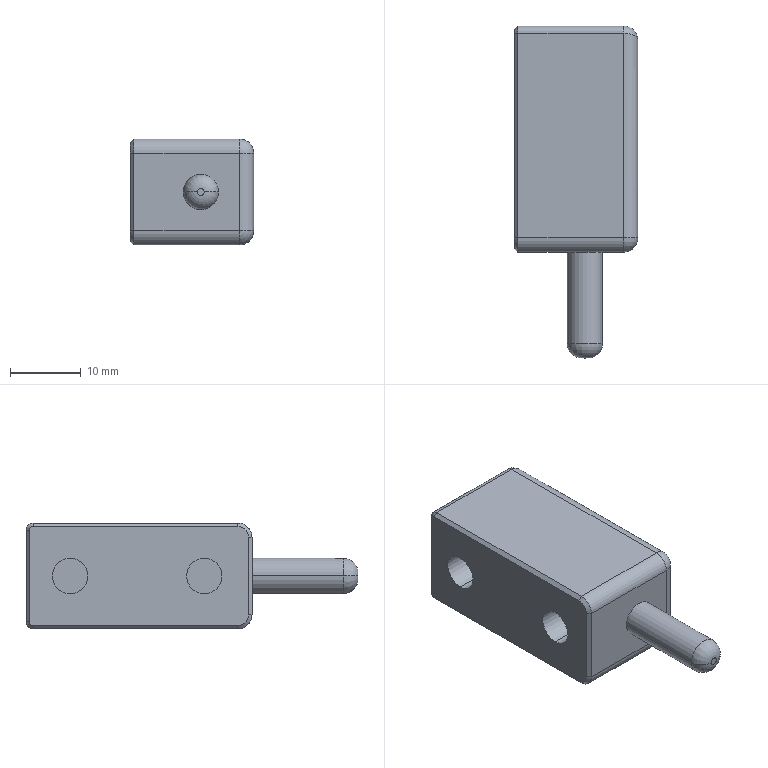Component | SolidWorks | LeftDoorPanelAssembly-1_CL203-2-A-1 | 1 solid | 37 faces | box 17.5 x 47 x 15 mm | volume 7950 mm3 | cylinder 14 | plane 13 | cone 4 | torus 2 | spline 2 | sphere 2 | commonest cylinder face diameters 5 x6 4 x6 2 x2
STEP:
#1=COLOUR_RGB('',0.7922,0.8196,0.9333);
#2=FILL_AREA_STYLE_COLOUR('',#1);
#3=FILL_AREA_STYLE('',(#2));
#4=SURFACE_STYLE_FILL_AREA(#3);
#5=SURFACE_SIDE_STYLE('',(#4));
#6=SURFACE_STYLE_USAGE(.BOTH.,#5);
#7=PRESENTATION_STYLE_ASSIGNMENT((#6));
#8=CARTESIAN_POINT('',(20.575,-3.877,-2.386));
#9=VERTEX_POINT('',#8);
#10=CARTESIAN_POINT('',(20.378,-3.877,-2.386));
#11=VERTEX_POINT('',#10);
#12=CARTESIAN_POINT('',(20.477,-3.877,-2.386));
#13=DIRECTION('',(-0.,1.,0.));
#14=DIRECTION('',(-1.,-0.,-0.));
#15=AXIS2_PLACEMENT_3D('',#12,#13,#14);
#16=CIRCLE('',#15,0.09843);
#17=EDGE_CURVE('',#9,#11,#16,.T.);
#18=ORIENTED_EDGE('',*,*,#17,.F.);
#19=CARTESIAN_POINT('',(20.496,-3.956,-2.386));
#20=VERTEX_POINT('',#19);
#21=CARTESIAN_POINT('',(20.496,-3.877,-2.386));
#22=DIRECTION('',(0.,0.,-1.));
#23=DIRECTION('',(-1.,0.,-0.));
#24=AXIS2_PLACEMENT_3D('',#21,#22,#23);
#25=CIRCLE('',#24,0.07874);
#26=EDGE_CURVE('',#9,#20,#25,.T.);
#27=ORIENTED_EDGE('',*,*,#26,.T.);
#28=CARTESIAN_POINT('',(20.457,-3.956,-2.386));
#29=VERTEX_POINT('',#28);
#30=CARTESIAN_POINT('',(20.477,-3.956,-2.386));
#31=DIRECTION('',(0.,-1.,-0.));
#32=DIRECTION('',(-1.,0.,-0.));
#33=AXIS2_PLACEMENT_3D('',#30,#31,#32);
#34=CIRCLE('',#33,0.01969);
#35=EDGE_CURVE('',#29,#20,#34,.T.);
#36=ORIENTED_EDGE('',*,*,#35,.F.);
#37=CARTESIAN_POINT('',(20.457,-3.877,-2.386));
#38=DIRECTION('',(-0.,-0.,1.));
#39=DIRECTION('',(1.,0.,0.));
#40=AXIS2_PLACEMENT_3D('',#37,#38,#39);
#41=CIRCLE('',#40,0.07874);
#42=EDGE_CURVE('',#11,#29,#41,.T.);
#43=ORIENTED_EDGE('',*,*,#42,.F.);
#44=EDGE_LOOP('',(#18,#27,#36,#43));
#45=FACE_OUTER_BOUND('',#44,.T.);
#46=CARTESIAN_POINT('',(20.477,-3.877,-2.386));
#47=DIRECTION('',(0.,-1.,-0.));
#48=DIRECTION('',(-1.,-0.,-0.));
#49=AXIS2_PLACEMENT_3D('',#46,#47,#48);
#50=TOROIDAL_SURFACE('',#49,0.01969,0.07874);
#51=ADVANCED_FACE('',(#45),#50,.T.);
#52=ORIENTED_EDGE('',*,*,#17,.T.);
#53=CARTESIAN_POINT('',(20.378,-3.365,-2.386));
#54=VERTEX_POINT('',#53);
#55=CARTESIAN_POINT('',(20.378,-3.956,-2.386));
#56=DIRECTION('',(-0.,1.,0.));
#57=VECTOR('',#56,39.37);
#58=LINE('',#55,#57);
#59=EDGE_CURVE('',#11,#54,#58,.T.);
#60=ORIENTED_EDGE('',*,*,#59,.T.);
#61=CARTESIAN_POINT('',(20.575,-3.365,-2.386));
#62=VERTEX_POINT('',#61);
#63=CARTESIAN_POINT('',(20.477,-3.365,-2.386));
#64=DIRECTION('',(0.,-1.,-0.));
#65=DIRECTION('',(1.,0.,0.));
#66=AXIS2_PLACEMENT_3D('',#63,#64,#65);
#67=CIRCLE('',#66,0.09843);
#68=EDGE_CURVE('',#54,#62,#67,.T.);
#69=ORIENTED_EDGE('',*,*,#68,.T.);
#70=CARTESIAN_POINT('',(20.575,-3.956,-2.386));
#71=DIRECTION('',(-0.,1.,0.));
#72=VECTOR('',#71,39.37);
#73=LINE('',#70,#72);
#74=EDGE_CURVE('',#9,#62,#73,.T.);
#75=ORIENTED_EDGE('',*,*,#74,.F.);
#76=EDGE_LOOP('',(#52,#60,#69,#75));
#77=FACE_OUTER_BOUND('',#76,.T.);
#78=CARTESIAN_POINT('',(20.477,-3.956,-2.386));
#79=DIRECTION('',(-0.,1.,0.));
#80=DIRECTION('',(1.,0.,0.));
#81=AXIS2_PLACEMENT_3D('',#78,#79,#80);
#82=CYLINDRICAL_SURFACE('',#81,0.09843);
#83=ADVANCED_FACE('',(#77),#82,.T.);
#84=CARTESIAN_POINT('',(20.083,-3.1,-2.287));
#85=VERTEX_POINT('',#84);
#86=CARTESIAN_POINT('',(20.083,-3.1,-2.484));
#87=VERTEX_POINT('',#86);
#88=CARTESIAN_POINT('',(20.083,-3.1,-2.386));
#89=DIRECTION('',(-1.,-0.,-0.));
#90=DIRECTION('',(0.,0.,-1.));
#91=AXIS2_PLACEMENT_3D('',#88,#89,#90);
#92=CIRCLE('',#91,0.09843);
#93=EDGE_CURVE('',#85,#87,#92,.T.);
#94=ORIENTED_EDGE('',*,*,#93,.T.);
#95=CARTESIAN_POINT('',(20.693,-3.1,-2.484));
#96=VERTEX_POINT('',#95);
#97=CARTESIAN_POINT('',(20.083,-3.1,-2.484));
#98=DIRECTION('',(1.,0.,0.));
#99=VECTOR('',#98,39.37);
#100=LINE('',#97,#99);
#101=EDGE_CURVE('',#87,#96,#100,.T.);
#102=ORIENTED_EDGE('',*,*,#101,.T.);
#103=CARTESIAN_POINT('',(20.693,-3.1,-2.287));
#104=VERTEX_POINT('',#103);
#105=CARTESIAN_POINT('',(20.693,-3.1,-2.386));
#106=DIRECTION('',(1.,0.,0.));
#107=DIRECTION('',(0.,-0.,1.));
#108=AXIS2_PLACEMENT_3D('',#105,#106,#107);
#109=CIRCLE('',#108,0.09843);
#110=EDGE_CURVE('',#96,#104,#109,.T.);
#111=ORIENTED_EDGE('',*,*,#110,.T.);
#112=CARTESIAN_POINT('',(20.083,-3.1,-2.287));
#113=DIRECTION('',(1.,0.,0.));
#114=VECTOR('',#113,39.37);
#115=LINE('',#112,#114);
#116=EDGE_CURVE('',#85,#104,#115,.T.);
#117=ORIENTED_EDGE('',*,*,#116,.F.);
#118=EDGE_LOOP('',(#94,#102,#111,#117));
#119=FACE_OUTER_BOUND('',#118,.T.);
#120=CARTESIAN_POINT('',(20.083,-3.1,-2.386));
#121=DIRECTION('',(1.,0.,0.));
#122=DIRECTION('',(0.,-0.,1.));
#123=AXIS2_PLACEMENT_3D('',#120,#121,#122);
#124=CYLINDRICAL_SURFACE('',#123,0.09843);
#125=ADVANCED_FACE('',(#119),#124,.F.);
#126=CARTESIAN_POINT('',(20.083,-2.352,-2.287));
#127=VERTEX_POINT('',#126);
#128=CARTESIAN_POINT('',(20.083,-2.352,-2.484));
#129=VERTEX_POINT('',#128);
#130=CARTESIAN_POINT('',(20.083,-2.352,-2.386));
#131=DIRECTION('',(-1.,-0.,-0.));
#132=DIRECTION('',(0.,0.,-1.));
#133=AXIS2_PLACEMENT_3D('',#130,#131,#132);
#134=CIRCLE('',#133,0.09843);
#135=EDGE_CURVE('',#127,#129,#134,.T.);
#136=ORIENTED_EDGE('',*,*,#135,.T.);
#137=CARTESIAN_POINT('',(20.693,-2.352,-2.484));
#138=VERTEX_POINT('',#137);
#139=CARTESIAN_POINT('',(20.083,-2.352,-2.484));
#140=DIRECTION('',(1.,0.,0.));
#141=VECTOR('',#140,39.37);
#142=LINE('',#139,#141);
#143=EDGE_CURVE('',#129,#138,#142,.T.);
#144=ORIENTED_EDGE('',*,*,#143,.T.);
#145=CARTESIAN_POINT('',(20.693,-2.352,-2.287));
#146=VERTEX_POINT('',#145);
#147=CARTESIAN_POINT('',(20.693,-2.352,-2.386));
#148=DIRECTION('',(1.,0.,0.));
#149=DIRECTION('',(0.,-0.,1.));
#150=AXIS2_PLACEMENT_3D('',#147,#148,#149);
#151=CIRCLE('',#150,0.09843);
#152=EDGE_CURVE('',#138,#146,#151,.T.);
#153=ORIENTED_EDGE('',*,*,#152,.T.);
#154=CARTESIAN_POINT('',(20.083,-2.352,-2.287));
#155=DIRECTION('',(1.,0.,0.));
#156=VECTOR('',#155,39.37);
#157=LINE('',#154,#156);
#158=EDGE_CURVE('',#127,#146,#157,.T.);
#159=ORIENTED_EDGE('',*,*,#158,.F.);
#160=EDGE_LOOP('',(#136,#144,#153,#159));
#161=FACE_OUTER_BOUND('',#160,.T.);
#162=CARTESIAN_POINT('',(20.083,-2.352,-2.386));
#163=DIRECTION('',(1.,0.,0.));
#164=DIRECTION('',(0.,-0.,1.));
#165=AXIS2_PLACEMENT_3D('',#162,#163,#164);
#166=CYLINDRICAL_SURFACE('',#165,0.09843);
#167=ADVANCED_FACE('',(#161),#166,.F.);
#168=ORIENTED_EDGE('',*,*,#143,.F.);
#169=CARTESIAN_POINT('',(20.083,-2.352,-2.386));
#170=DIRECTION('',(-1.,-0.,-0.));
#171=DIRECTION('',(0.,0.,-1.));
#172=AXIS2_PLACEMENT_3D('',#169,#170,#171);
#173=CIRCLE('',#172,0.09843);
#174=EDGE_CURVE('',#129,#127,#173,.T.);
#175=ORIENTED_EDGE('',*,*,#174,.T.);
#176=ORIENTED_EDGE('',*,*,#158,.T.);
#177=CARTESIAN_POINT('',(20.693,-2.352,-2.386));
#178=DIRECTION('',(1.,0.,0.));
#179=DIRECTION('',(0.,-0.,1.));
#180=AXIS2_PLACEMENT_3D('',#177,#178,#179);
#181=CIRCLE('',#180,0.09843);
#182=EDGE_CURVE('',#146,#138,#181,.T.);
#183=ORIENTED_EDGE('',*,*,#182,.T.);
#184=EDGE_LOOP('',(#168,#175,#176,#183));
#185=FACE_OUTER_BOUND('',#184,.T.);
#186=CARTESIAN_POINT('',(20.083,-2.352,-2.386));
#187=DIRECTION('',(1.,0.,0.));
#188=DIRECTION('',(0.,-0.,1.));
#189=AXIS2_PLACEMENT_3D('',#186,#187,#188);
#190=CYLINDRICAL_SURFACE('',#189,0.09843);
#191=ADVANCED_FACE('',(#185),#190,.F.);
#192=ORIENTED_EDGE('',*,*,#101,.F.);
#193=CARTESIAN_POINT('',(20.083,-3.1,-2.386));
#194=DIRECTION('',(-1.,-0.,-0.));
#195=DIRECTION('',(0.,0.,-1.));
#196=AXIS2_PLACEMENT_3D('',#193,#194,#195);
#197=CIRCLE('',#196,0.09843);
#198=EDGE_CURVE('',#87,#85,#197,.T.);
#199=ORIENTED_EDGE('',*,*,#198,.T.);
#200=ORIENTED_EDGE('',*,*,#116,.T.);
#201=CARTESIAN_POINT('',(20.693,-3.1,-2.386));
#202=DIRECTION('',(1.,0.,0.));
#203=DIRECTION('',(0.,-0.,1.));
#204=AXIS2_PLACEMENT_3D('',#201,#202,#203);
#205=CIRCLE('',#204,0.09843);
#206=EDGE_CURVE('',#104,#96,#205,.T.);
#207=ORIENTED_EDGE('',*,*,#206,.T.);
#208=EDGE_LOOP('',(#192,#199,#200,#207));
#209=FACE_OUTER_BOUND('',#208,.T.);
#210=CARTESIAN_POINT('',(20.083,-3.1,-2.386));
#211=DIRECTION('',(1.,0.,0.));
#212=DIRECTION('',(0.,-0.,1.));
#213=AXIS2_PLACEMENT_3D('',#210,#211,#212);
#214=CYLINDRICAL_SURFACE('',#213,0.09843);
#215=ADVANCED_FACE('',(#209),#214,.F.);
#216=CARTESIAN_POINT('',(20.693,-3.365,-2.169));
#217=VERTEX_POINT('',#216);
#218=CARTESIAN_POINT('',(20.103,-3.365,-2.169));
#219=VERTEX_POINT('',#218);
#220=CARTESIAN_POINT('',(20.083,-3.365,-2.169));
#221=DIRECTION('',(-1.,-0.,-0.));
#222=VECTOR('',#221,39.37);
#223=LINE('',#220,#222);
#224=EDGE_CURVE('',#217,#219,#223,.T.);
#225=ORIENTED_EDGE('',*,*,#224,.T.);
#226=CARTESIAN_POINT('',(20.103,-3.365,-2.602));
#227=VERTEX_POINT('',#226);
#228=CARTESIAN_POINT('',(20.103,-3.365,-2.602));
#229=DIRECTION('',(0.,0.,-1.));
#230=VECTOR('',#229,39.37);
#231=LINE('',#228,#230);
#232=EDGE_CURVE('',#219,#227,#231,.T.);
#233=ORIENTED_EDGE('',*,*,#232,.T.);
#234=CARTESIAN_POINT('',(20.693,-3.365,-2.602));
#235=VERTEX_POINT('',#234);
#236=CARTESIAN_POINT('',(20.083,-3.365,-2.602));
#237=DIRECTION('',(1.,0.,0.));
#238=VECTOR('',#237,39.37);
#239=LINE('',#236,#238);
#240=EDGE_CURVE('',#227,#235,#239,.T.);
#241=ORIENTED_EDGE('',*,*,#240,.T.);
#242=CARTESIAN_POINT('',(20.693,-3.365,-2.091));
#243=DIRECTION('',(-0.,-0.,1.));
#244=VECTOR('',#243,39.37);
#245=LINE('',#242,#244);
#246=EDGE_CURVE('',#235,#217,#245,.T.);
#247=ORIENTED_EDGE('',*,*,#246,.T.);
#248=EDGE_LOOP('',(#225,#233,#241,#247));
#249=FACE_OUTER_BOUND('',#248,.T.);
#250=CARTESIAN_POINT('',(20.477,-3.365,-2.386));
#251=DIRECTION('',(0.,-1.,-0.));
#252=DIRECTION('',(1.,0.,0.));
#253=AXIS2_PLACEMENT_3D('',#250,#251,#252);
#254=CIRCLE('',#253,0.09843);
#255=EDGE_CURVE('',#62,#54,#254,.T.);
#256=ORIENTED_EDGE('',*,*,#255,.F.);
#257=ORIENTED_EDGE('',*,*,#68,.F.);
#258=EDGE_LOOP('',(#256,#257));
#259=FACE_BOUND('',#258,.T.);
#260=CARTESIAN_POINT('',(20.083,-3.365,-2.091));
#261=DIRECTION('',(-0.,1.,0.));
#262=DIRECTION('',(1.,0.,0.));
#263=AXIS2_PLACEMENT_3D('',#260,#261,#262);
#264=PLANE('',#263);
#265=ADVANCED_FACE('',(#249,#259),#264,.F.);
#266=CARTESIAN_POINT('',(20.083,-3.346,-2.169));
#267=VERTEX_POINT('',#266);
#268=CARTESIAN_POINT('',(20.083,-3.287,-2.11));
#269=VERTEX_POINT('',#268);
#270=CARTESIAN_POINT('',(20.083,-3.287,-2.169));
#271=DIRECTION('',(-1.,-0.,-0.));
#272=DIRECTION('',(0.,0.,-1.));
#273=AXIS2_PLACEMENT_3D('',#270,#271,#272);
#274=CIRCLE('',#273,0.05906);
#275=EDGE_CURVE('',#267,#269,#274,.T.);
#276=ORIENTED_EDGE('',*,*,#275,.T.);
#277=CARTESIAN_POINT('',(20.083,-2.145,-2.11));
#278=VERTEX_POINT('',#277);
#279=CARTESIAN_POINT('',(20.083,-2.145,-2.11));
#280=DIRECTION('',(-0.,1.,0.));
#281=VECTOR('',#280,39.37);
#282=LINE('',#279,#281);
#283=EDGE_CURVE('',#269,#278,#282,.T.);
#284=ORIENTED_EDGE('',*,*,#283,.T.);
#285=CARTESIAN_POINT('',(20.083,-2.125,-2.13));
#286=VERTEX_POINT('',#285);
#287=CARTESIAN_POINT('',(20.083,-2.145,-2.13));
#288=DIRECTION('',(-1.,-0.,-0.));
#289=DIRECTION('',(0.,0.,-1.));
#290=AXIS2_PLACEMENT_3D('',#287,#288,#289);
#291=CIRCLE('',#290,0.01969);
#292=EDGE_CURVE('',#278,#286,#291,.T.);
#293=ORIENTED_EDGE('',*,*,#292,.T.);
#294=CARTESIAN_POINT('',(20.083,-2.125,-2.642));
#295=VERTEX_POINT('',#294);
#296=CARTESIAN_POINT('',(20.083,-2.125,-2.642));
#297=DIRECTION('',(0.,0.,-1.));
#298=VECTOR('',#297,39.37);
#299=LINE('',#296,#298);
#300=EDGE_CURVE('',#286,#295,#299,.T.);
#301=ORIENTED_EDGE('',*,*,#300,.T.);
#302=CARTESIAN_POINT('',(20.083,-2.145,-2.661));
#303=VERTEX_POINT('',#302);
#304=CARTESIAN_POINT('',(20.083,-2.145,-2.642));
#305=DIRECTION('',(-1.,-0.,-0.));
#306=DIRECTION('',(0.,0.,-1.));
#307=AXIS2_PLACEMENT_3D('',#304,#305,#306);
#308=CIRCLE('',#307,0.01969);
#309=EDGE_CURVE('',#295,#303,#308,.T.);
#310=ORIENTED_EDGE('',*,*,#309,.T.);
#311=CARTESIAN_POINT('',(20.083,-3.287,-2.661));
#312=VERTEX_POINT('',#311);
#313=CARTESIAN_POINT('',(20.083,-3.287,-2.661));
#314=DIRECTION('',(0.,-1.,-0.));
#315=VECTOR('',#314,39.37);
#316=LINE('',#313,#315);
#317=EDGE_CURVE('',#303,#312,#316,.T.);
#318=ORIENTED_EDGE('',*,*,#317,.T.);
#319=CARTESIAN_POINT('',(20.083,-3.346,-2.602));
#320=VERTEX_POINT('',#319);
#321=CARTESIAN_POINT('',(20.083,-3.287,-2.602));
#322=DIRECTION('',(-1.,-0.,-0.));
#323=DIRECTION('',(0.,0.,-1.));
#324=AXIS2_PLACEMENT_3D('',#321,#322,#323);
#325=CIRCLE('',#324,0.05906);
#326=EDGE_CURVE('',#312,#320,#325,.T.);
#327=ORIENTED_EDGE('',*,*,#326,.T.);
#328=CARTESIAN_POINT('',(20.083,-3.346,-2.169));
#329=DIRECTION('',(-0.,-0.,1.));
#330=VECTOR('',#329,39.37);
#331=LINE('',#328,#330);
#332=EDGE_CURVE('',#320,#267,#331,.T.);
#333=ORIENTED_EDGE('',*,*,#332,.T.);
#334=EDGE_LOOP('',(#276,#284,#293,#301,#310,#318,#327,#333));
#335=FACE_OUTER_BOUND('',#334,.T.);
#336=ORIENTED_EDGE('',*,*,#93,.F.);
#337=ORIENTED_EDGE('',*,*,#198,.F.);
#338=EDGE_LOOP('',(#336,#337));
#339=FACE_BOUND('',#338,.T.);
#340=ORIENTED_EDGE('',*,*,#135,.F.);
#341=ORIENTED_EDGE('',*,*,#174,.F.);
#342=EDGE_LOOP('',(#340,#341));
#343=FACE_BOUND('',#342,.T.);
#344=CARTESIAN_POINT('',(20.083,-2.145,-2.642));
#345=DIRECTION('',(-1.,-0.,-0.));
#346=DIRECTION('',(0.,0.,-1.));
#347=AXIS2_PLACEMENT_3D('',#344,#345,#346);
#348=PLANE('',#347);
#349=ADVANCED_FACE('',(#335,#339,#343),#348,.T.);
#350=CARTESIAN_POINT('',(20.772,-2.184,-2.169));
#351=VERTEX_POINT('',#350);
#352=CARTESIAN_POINT('',(20.772,-3.287,-2.169));
#353=VERTEX_POINT('',#352);
#354=CARTESIAN_POINT('',(20.772,-2.145,-2.169));
#355=DIRECTION('',(0.,-1.,-0.));
#356=VECTOR('',#355,39.37);
#357=LINE('',#354,#356);
#358=EDGE_CURVE('',#351,#353,#357,.T.);
#359=ORIENTED_EDGE('',*,*,#358,.T.);
#360=CARTESIAN_POINT('',(20.772,-3.287,-2.602));
#361=VERTEX_POINT('',#360);
#362=CARTESIAN_POINT('',(20.772,-3.287,-2.642));
#363=DIRECTION('',(0.,0.,-1.));
#364=VECTOR('',#363,39.37);
#365=LINE('',#362,#364);
#366=EDGE_CURVE('',#353,#361,#365,.T.);
#367=ORIENTED_EDGE('',*,*,#366,.T.);
#368=CARTESIAN_POINT('',(20.772,-2.184,-2.602));
#369=VERTEX_POINT('',#368);
#370=CARTESIAN_POINT('',(20.772,-2.145,-2.602));
#371=DIRECTION('',(-0.,1.,0.));
#372=VECTOR('',#371,39.37);
#373=LINE('',#370,#372);
#374=EDGE_CURVE('',#361,#369,#373,.T.);
#375=ORIENTED_EDGE('',*,*,#374,.T.);
#376=CARTESIAN_POINT('',(20.772,-2.184,-2.642));
#377=DIRECTION('',(-0.,-0.,1.));
#378=VECTOR('',#377,39.37);
#379=LINE('',#376,#378);
#380=EDGE_CURVE('',#369,#351,#379,.T.);
#381=ORIENTED_EDGE('',*,*,#380,.T.);
#382=EDGE_LOOP('',(#359,#367,#375,#381));
#383=FACE_OUTER_BOUND('',#382,.T.);
#384=CARTESIAN_POINT('',(20.772,-2.145,-2.642));
#385=DIRECTION('',(-1.,-0.,-0.));
#386=DIRECTION('',(0.,0.,-1.));
#387=AXIS2_PLACEMENT_3D('',#384,#385,#386);
#388=PLANE('',#387);
#389=ADVANCED_FACE('',(#383),#388,.F.);
#390=CARTESIAN_POINT('',(20.103,-2.145,-2.091));
#391=VERTEX_POINT('',#390);
#392=CARTESIAN_POINT('',(20.693,-2.145,-2.091));
#393=VERTEX_POINT('',#392);
#394=CARTESIAN_POINT('',(20.083,-2.145,-2.091));
#395=DIRECTION('',(1.,0.,0.));
#396=VECTOR('',#395,39.37);
#397=LINE('',#394,#396);
#398=EDGE_CURVE('',#391,#393,#397,.T.);
#399=ORIENTED_EDGE('',*,*,#398,.F.);
#400=CARTESIAN_POINT('',(20.103,-3.287,-2.091));
#401=VERTEX_POINT('',#400);
#402=CARTESIAN_POINT('',(20.103,-3.287,-2.091));
#403=DIRECTION('',(0.,-1.,-0.));
#404=VECTOR('',#403,39.37);
#405=LINE('',#402,#404);
#406=EDGE_CURVE('',#391,#401,#405,.T.);
#407=ORIENTED_EDGE('',*,*,#406,.T.);
#408=CARTESIAN_POINT('',(20.693,-3.287,-2.091));
#409=VERTEX_POINT('',#408);
#410=CARTESIAN_POINT('',(20.083,-3.287,-2.091));
#411=DIRECTION('',(1.,0.,0.));
#412=VECTOR('',#411,39.37);
#413=LINE('',#410,#412);
#414=EDGE_CURVE('',#401,#409,#413,.T.);
#415=ORIENTED_EDGE('',*,*,#414,.T.);
#416=CARTESIAN_POINT('',(20.693,-3.365,-2.091));
#417=DIRECTION('',(-0.,1.,0.));
#418=VECTOR('',#417,39.37);
#419=LINE('',#416,#418);
#420=EDGE_CURVE('',#409,#393,#419,.T.);
#421=ORIENTED_EDGE('',*,*,#420,.T.);
#422=EDGE_LOOP('',(#399,#407,#415,#421));
#423=FACE_OUTER_BOUND('',#422,.T.);
#424=CARTESIAN_POINT('',(20.083,-3.365,-2.091));
#425=DIRECTION('',(0.,0.,-1.));
#426=DIRECTION('',(1.,0.,0.));
#427=AXIS2_PLACEMENT_3D('',#424,#425,#426);
#428=PLANE('',#427);
#429=ADVANCED_FACE('',(#423),#428,.F.);
#430=CARTESIAN_POINT('',(20.103,-2.105,-2.13));
#431=VERTEX_POINT('',#430);
#432=CARTESIAN_POINT('',(20.693,-2.105,-2.13));
#433=VERTEX_POINT('',#432);
#434=CARTESIAN_POINT('',(20.083,-2.105,-2.13));
#435=DIRECTION('',(1.,0.,0.));
#436=VECTOR('',#435,39.37);
#437=LINE('',#434,#436);
#438=EDGE_CURVE('',#431,#433,#437,.T.);
#439=ORIENTED_EDGE('',*,*,#438,.F.);
#440=CARTESIAN_POINT('',(20.103,-2.145,-2.13));
#441=DIRECTION('',(1.,0.,0.));
#442=DIRECTION('',(0.,0.,-1.));
#443=AXIS2_PLACEMENT_3D('',#440,#441,#442);
#444=CIRCLE('',#443,0.03937);
#445=EDGE_CURVE('',#431,#391,#444,.T.);
#446=ORIENTED_EDGE('',*,*,#445,.T.);
#447=ORIENTED_EDGE('',*,*,#398,.T.);
#448=CARTESIAN_POINT('',(20.693,-2.145,-2.13));
#449=DIRECTION('',(-1.,-0.,-0.));
#450=DIRECTION('',(0.,0.,-1.));
#451=AXIS2_PLACEMENT_3D('',#448,#449,#450);
#452=CIRCLE('',#451,0.03937);
#453=EDGE_CURVE('',#393,#433,#452,.T.);
#454=ORIENTED_EDGE('',*,*,#453,.T.);
#455=EDGE_LOOP('',(#439,#446,#447,#454));
#456=FACE_OUTER_BOUND('',#455,.T.);
#457=CARTESIAN_POINT('',(20.083,-2.145,-2.13));
#458=DIRECTION('',(1.,0.,0.));
#459=DIRECTION('',(0.,-0.,1.));
#460=AXIS2_PLACEMENT_3D('',#457,#458,#459);
#461=CYLINDRICAL_SURFACE('',#460,0.03937);
#462=ADVANCED_FACE('',(#456),#461,.T.);
#463=CARTESIAN_POINT('',(20.103,-2.105,-2.642));
#464=VERTEX_POINT('',#463);
#465=CARTESIAN_POINT('',(20.693,-2.105,-2.642));
#466=VERTEX_POINT('',#465);
#467=CARTESIAN_POINT('',(20.083,-2.105,-2.642));
#468=DIRECTION('',(1.,0.,0.));
#469=VECTOR('',#468,39.37);
#470=LINE('',#467,#469);
#471=EDGE_CURVE('',#464,#466,#470,.T.);
#472=ORIENTED_EDGE('',*,*,#471,.F.);
#473=CARTESIAN_POINT('',(20.103,-2.105,-2.13));
#474=DIRECTION('',(-0.,-0.,1.));
#475=VECTOR('',#474,39.37);
#476=LINE('',#473,#475);
#477=EDGE_CURVE('',#464,#431,#476,.T.);
#478=ORIENTED_EDGE('',*,*,#477,.T.);
#479=ORIENTED_EDGE('',*,*,#438,.T.);
#480=CARTESIAN_POINT('',(20.693,-2.105,-2.13));
#481=DIRECTION('',(0.,0.,-1.));
#482=VECTOR('',#481,39.37);
#483=LINE('',#480,#482);
#484=EDGE_CURVE('',#433,#466,#483,.T.);
#485=ORIENTED_EDGE('',*,*,#484,.T.);
#486=EDGE_LOOP('',(#472,#478,#479,#485));
#487=FACE_OUTER_BOUND('',#486,.T.);
#488=CARTESIAN_POINT('',(20.083,-2.105,-2.13));
#489=DIRECTION('',(0.,-1.,-0.));
#490=DIRECTION('',(-1.,-0.,-0.));
#491=AXIS2_PLACEMENT_3D('',#488,#489,#490);
#492=PLANE('',#491);
#493=ADVANCED_FACE('',(#487),#492,.F.);
#494=CARTESIAN_POINT('',(20.103,-2.145,-2.681));
#495=VERTEX_POINT('',#494);
#496=CARTESIAN_POINT('',(20.693,-2.145,-2.681));
#497=VERTEX_POINT('',#496);
#498=CARTESIAN_POINT('',(20.083,-2.145,-2.681));
#499=DIRECTION('',(1.,0.,0.));
#500=VECTOR('',#499,39.37);
#501=LINE('',#498,#500);
#502=EDGE_CURVE('',#495,#497,#501,.T.);
#503=ORIENTED_EDGE('',*,*,#502,.F.);
#504=CARTESIAN_POINT('',(20.103,-2.145,-2.642));
#505=DIRECTION('',(1.,0.,0.));
#506=DIRECTION('',(0.,0.,-1.));
#507=AXIS2_PLACEMENT_3D('',#504,#505,#506);
#508=CIRCLE('',#507,0.03937);
#509=EDGE_CURVE('',#495,#464,#508,.T.);
#510=ORIENTED_EDGE('',*,*,#509,.T.);
#511=ORIENTED_EDGE('',*,*,#471,.T.);
#512=CARTESIAN_POINT('',(20.693,-2.145,-2.642));
#513=DIRECTION('',(-1.,-0.,-0.));
#514=DIRECTION('',(0.,0.,-1.));
#515=AXIS2_PLACEMENT_3D('',#512,#513,#514);
#516=CIRCLE('',#515,0.03937);
#517=EDGE_CURVE('',#466,#497,#516,.T.);
#518=ORIENTED_EDGE('',*,*,#517,.T.);
#519=EDGE_LOOP('',(#503,#510,#511,#518));
#520=FACE_OUTER_BOUND('',#519,.T.);
#521=CARTESIAN_POINT('',(20.083,-2.145,-2.642));
#522=DIRECTION('',(1.,0.,0.));
#523=DIRECTION('',(0.,-0.,1.));
#524=AXIS2_PLACEMENT_3D('',#521,#522,#523);
#525=CYLINDRICAL_SURFACE('',#524,0.03937);
#526=ADVANCED_FACE('',(#520),#525,.T.);
#527=CARTESIAN_POINT('',(20.693,-3.287,-2.681));
#528=VERTEX_POINT('',#527);
#529=CARTESIAN_POINT('',(20.103,-3.287,-2.681));
#530=VERTEX_POINT('',#529);
#531=CARTESIAN_POINT('',(20.083,-3.287,-2.681));
#532=DIRECTION('',(-1.,-0.,-0.));
#533=VECTOR('',#532,39.37);
#534=LINE('',#531,#533);
#535=EDGE_CURVE('',#528,#530,#534,.T.);
#536=ORIENTED_EDGE('',*,*,#535,.T.);
#537=CARTESIAN_POINT('',(20.103,-2.145,-2.681));
#538=DIRECTION('',(-0.,1.,0.));
#539=VECTOR('',#538,39.37);
#540=LINE('',#537,#539);
#541=EDGE_CURVE('',#530,#495,#540,.T.);
#542=ORIENTED_EDGE('',*,*,#541,.T.);
#543=ORIENTED_EDGE('',*,*,#502,.T.);
#544=CARTESIAN_POINT('',(20.693,-2.145,-2.681));
#545=DIRECTION('',(0.,-1.,-0.));
#546=VECTOR('',#545,39.37);
#547=LINE('',#544,#546);
#548=EDGE_CURVE('',#497,#528,#547,.T.);
#549=ORIENTED_EDGE('',*,*,#548,.T.);
#550=EDGE_LOOP('',(#536,#542,#543,#549));
#551=FACE_OUTER_BOUND('',#550,.T.);
#552=CARTESIAN_POINT('',(20.083,-2.145,-2.681));
#553=DIRECTION('',(-0.,-0.,1.));
#554=DIRECTION('',(-1.,-0.,-0.));
#555=AXIS2_PLACEMENT_3D('',#552,#553,#554);
#556=PLANE('',#555);
#557=ADVANCED_FACE('',(#551),#556,.F.);
#558=ORIENTED_EDGE('',*,*,#420,.F.);
#559=CARTESIAN_POINT('',(20.693,-3.287,-2.169));
#560=DIRECTION('',(-0.,1.,0.));
#561=DIRECTION('',(1.,0.,0.));
#562=AXIS2_PLACEMENT_3D('',#559,#560,#561);
#563=CIRCLE('',#562,0.07874);
#564=EDGE_CURVE('',#409,#353,#563,.T.);
#565=ORIENTED_EDGE('',*,*,#564,.T.);
#566=ORIENTED_EDGE('',*,*,#358,.F.);
#567=CARTESIAN_POINT('',(20.693,-2.145,-2.091));
#568=CARTESIAN_POINT('',(20.739,-2.145,-2.091));
#569=CARTESIAN_POINT('',(20.772,-2.161,-2.123));
#570=CARTESIAN_POINT('',(20.772,-2.184,-2.169));
#571=(BOUNDED_CURVE()B_SPLINE_CURVE(3,(#567,#568,#569,#570),.UNSPECIFIED.,.F.,.F.)B_SPLINE_CURVE_WITH_KNOTS((4,4),(0.,1.571),.UNSPECIFIED.)CURVE()GEOMETRIC_REPRESENTATION_ITEM()RATIONAL_B_SPLINE_CURVE((1.,0.8047,0.8047,1.))REPRESENTATION_ITEM(''));
#572=EDGE_CURVE('',#393,#351,#571,.T.);
#573=ORIENTED_EDGE('',*,*,#572,.F.);
#574=EDGE_LOOP('',(#558,#565,#566,#573));
#575=FACE_OUTER_BOUND('',#574,.T.);
#576=CARTESIAN_POINT('',(20.693,-3.365,-2.169));
#577=DIRECTION('',(-0.,1.,0.));
#578=DIRECTION('',(1.,0.,0.));
#579=AXIS2_PLACEMENT_3D('',#576,#577,#578);
#580=CYLINDRICAL_SURFACE('',#579,0.07874);
#581=ADVANCED_FACE('',(#575),#580,.T.);
#582=ORIENTED_EDGE('',*,*,#453,.F.);
#583=ORIENTED_EDGE('',*,*,#572,.T.);
#584=CARTESIAN_POINT('',(20.693,-2.105,-2.13));
#585=CARTESIAN_POINT('',(20.739,-2.105,-2.13));
#586=CARTESIAN_POINT('',(20.772,-2.138,-2.146));
#587=CARTESIAN_POINT('',(20.772,-2.184,-2.169));
#588=(BOUNDED_CURVE()B_SPLINE_CURVE(3,(#584,#585,#586,#587),.UNSPECIFIED.,.F.,.T.)B_SPLINE_CURVE_WITH_KNOTS((4,4),(0.,1.571),.UNSPECIFIED.)CURVE()GEOMETRIC_REPRESENTATION_ITEM()RATIONAL_B_SPLINE_CURVE((1.,0.8047,0.8047,1.))REPRESENTATION_ITEM(''));
#589=EDGE_CURVE('',#433,#351,#588,.T.);
#590=ORIENTED_EDGE('',*,*,#589,.F.);
#591=EDGE_LOOP('',(#582,#583,#590));
#592=FACE_OUTER_BOUND('',#591,.T.);
#593=CARTESIAN_POINT('',(20.693,-2.145,-2.091));
#594=CARTESIAN_POINT('',(20.693,-2.105,-2.091));
#595=CARTESIAN_POINT('',(20.693,-2.105,-2.13));
#596=CARTESIAN_POINT('',(20.698,-2.145,-2.091));
#597=CARTESIAN_POINT('',(20.701,-2.105,-2.091));
#598=CARTESIAN_POINT('',(20.698,-2.105,-2.13));
#599=CARTESIAN_POINT('',(20.704,-2.145,-2.091));
#600=CARTESIAN_POINT('',(20.709,-2.106,-2.092));
#601=CARTESIAN_POINT('',(20.704,-2.106,-2.13));
#602=CARTESIAN_POINT('',(20.714,-2.146,-2.093));
#603=CARTESIAN_POINT('',(20.723,-2.11,-2.095));
#604=CARTESIAN_POINT('',(20.714,-2.108,-2.131));
#605=CARTESIAN_POINT('',(20.719,-2.147,-2.095));
#606=CARTESIAN_POINT('',(20.729,-2.113,-2.098));
#607=CARTESIAN_POINT('',(20.719,-2.109,-2.132));
#608=CARTESIAN_POINT('',(20.728,-2.149,-2.099));
#609=CARTESIAN_POINT('',(20.74,-2.119,-2.104));
#610=CARTESIAN_POINT('',(20.728,-2.113,-2.134));
#611=CARTESIAN_POINT('',(20.733,-2.15,-2.101));
#612=CARTESIAN_POINT('',(20.745,-2.123,-2.108));
#613=CARTESIAN_POINT('',(20.733,-2.116,-2.135));
#614=CARTESIAN_POINT('',(20.741,-2.153,-2.107));
#615=CARTESIAN_POINT('',(20.752,-2.13,-2.115));
#616=CARTESIAN_POINT('',(20.741,-2.122,-2.138));
#617=CARTESIAN_POINT('',(20.745,-2.155,-2.11));
#618=CARTESIAN_POINT('',(20.756,-2.134,-2.119));
#619=CARTESIAN_POINT('',(20.745,-2.125,-2.14));
#620=CARTESIAN_POINT('',(20.756,-2.16,-2.121));
#621=CARTESIAN_POINT('',(20.763,-2.145,-2.13));
#622=CARTESIAN_POINT('',(20.756,-2.136,-2.145));
#623=CARTESIAN_POINT('',(20.762,-2.164,-2.13));
#624=CARTESIAN_POINT('',(20.767,-2.153,-2.138));
#625=CARTESIAN_POINT('',(20.762,-2.145,-2.149));
#626=CARTESIAN_POINT('',(20.77,-2.174,-2.149));
#627=CARTESIAN_POINT('',(20.771,-2.169,-2.154));
#628=CARTESIAN_POINT('',(20.77,-2.164,-2.159));
#629=CARTESIAN_POINT('',(20.772,-2.179,-2.159));
#630=CARTESIAN_POINT('',(20.772,-2.176,-2.162));
#631=CARTESIAN_POINT('',(20.772,-2.174,-2.164));
#632=CARTESIAN_POINT('',(20.772,-2.184,-2.169));
#633=CARTESIAN_POINT('',(20.772,-2.184,-2.169));
#634=CARTESIAN_POINT('',(20.772,-2.184,-2.169));
#635=(BOUNDED_SURFACE()B_SPLINE_SURFACE(3,2,((#593,#594,#595),(#596,#597,#598),(#599,#600,#601),(#602,#603,#604),(#605,#606,#607),(#608,#609,#610),(#611,#612,#613),(#614,#615,#616),(#617,#618,#619),(#620,#621,#622),(#623,#624,#625),(#626,#627,#628),(#629,#630,#631),(#632,#633,#634)),.UNSPECIFIED.,.F.,.F.,.F.)B_SPLINE_SURFACE_WITH_KNOTS((4,2,2,2,2,2,4),(3,3),(6.283,6.48,6.676,6.872,7.069,7.461,7.854),(0.,1.),.UNSPECIFIED.)GEOMETRIC_REPRESENTATION_ITEM()RATIONAL_B_SPLINE_SURFACE(((1.,0.7071,1.),(1.,0.7071,1.),(1.,0.7117,1.),(1.,0.7291,1.),(1.,0.7418,1.),(1.,0.7724,1.),(1.,0.7902,1.),(1.,0.8276,1.),(1.,0.8471,1.),(1.,0.9038,1.),(1.,0.9387,1.),(1.,0.9867,1.),(1.,1.,1.),(1.,1.,1.)))REPRESENTATION_ITEM('')SURFACE());
#636=ADVANCED_FACE('',(#592),#635,.T.);
#637=ORIENTED_EDGE('',*,*,#589,.T.);
#638=ORIENTED_EDGE('',*,*,#380,.F.);
#639=CARTESIAN_POINT('',(20.693,-2.105,-2.642));
#640=CARTESIAN_POINT('',(20.739,-2.105,-2.642));
#641=CARTESIAN_POINT('',(20.772,-2.138,-2.625));
#642=CARTESIAN_POINT('',(20.772,-2.184,-2.602));
#643=(BOUNDED_CURVE()B_SPLINE_CURVE(3,(#639,#640,#641,#642),.UNSPECIFIED.,.F.,.F.)B_SPLINE_CURVE_WITH_KNOTS((4,4),(0.,1.571),.UNSPECIFIED.)CURVE()GEOMETRIC_REPRESENTATION_ITEM()RATIONAL_B_SPLINE_CURVE((1.,0.8047,0.8047,1.))REPRESENTATION_ITEM(''));
#644=EDGE_CURVE('',#466,#369,#643,.T.);
#645=ORIENTED_EDGE('',*,*,#644,.F.);
#646=ORIENTED_EDGE('',*,*,#484,.F.);
#647=EDGE_LOOP('',(#637,#638,#645,#646));
#648=FACE_OUTER_BOUND('',#647,.T.);
#649=CARTESIAN_POINT('',(20.693,-2.184,-2.13));
#650=DIRECTION('',(0.,0.,-1.));
#651=DIRECTION('',(1.,0.,0.));
#652=AXIS2_PLACEMENT_3D('',#649,#650,#651);
#653=CYLINDRICAL_SURFACE('',#652,0.07874);
#654=ADVANCED_FACE('',(#648),#653,.T.);
#655=ORIENTED_EDGE('',*,*,#517,.F.);
#656=ORIENTED_EDGE('',*,*,#644,.T.);
#657=CARTESIAN_POINT('',(20.693,-2.145,-2.681));
#658=CARTESIAN_POINT('',(20.739,-2.145,-2.681));
#659=CARTESIAN_POINT('',(20.772,-2.161,-2.648));
#660=CARTESIAN_POINT('',(20.772,-2.184,-2.602));
#661=(BOUNDED_CURVE()B_SPLINE_CURVE(3,(#657,#658,#659,#660),.UNSPECIFIED.,.F.,.T.)B_SPLINE_CURVE_WITH_KNOTS((4,4),(-0.,1.571),.UNSPECIFIED.)CURVE()GEOMETRIC_REPRESENTATION_ITEM()RATIONAL_B_SPLINE_CURVE((1.,0.8047,0.8047,1.))REPRESENTATION_ITEM(''));
#662=EDGE_CURVE('',#497,#369,#661,.T.);
#663=ORIENTED_EDGE('',*,*,#662,.F.);
#664=EDGE_LOOP('',(#655,#656,#663));
#665=FACE_OUTER_BOUND('',#664,.T.);
#666=CARTESIAN_POINT('',(20.693,-2.105,-2.642));
#667=CARTESIAN_POINT('',(20.693,-2.105,-2.681));
#668=CARTESIAN_POINT('',(20.693,-2.145,-2.681));
#669=CARTESIAN_POINT('',(20.698,-2.105,-2.642));
#670=CARTESIAN_POINT('',(20.701,-2.105,-2.681));
#671=CARTESIAN_POINT('',(20.698,-2.145,-2.681));
#672=CARTESIAN_POINT('',(20.704,-2.106,-2.641));
#673=CARTESIAN_POINT('',(20.709,-2.106,-2.68));
#674=CARTESIAN_POINT('',(20.704,-2.145,-2.681));
#675=CARTESIAN_POINT('',(20.714,-2.108,-2.64));
#676=CARTESIAN_POINT('',(20.723,-2.11,-2.676));
#677=CARTESIAN_POINT('',(20.714,-2.146,-2.679));
#678=CARTESIAN_POINT('',(20.719,-2.109,-2.64));
#679=CARTESIAN_POINT('',(20.729,-2.113,-2.674));
#680=CARTESIAN_POINT('',(20.719,-2.147,-2.677));
#681=CARTESIAN_POINT('',(20.728,-2.113,-2.638));
#682=CARTESIAN_POINT('',(20.74,-2.119,-2.667));
#683=CARTESIAN_POINT('',(20.728,-2.149,-2.673));
#684=CARTESIAN_POINT('',(20.733,-2.116,-2.637));
#685=CARTESIAN_POINT('',(20.745,-2.123,-2.664));
#686=CARTESIAN_POINT('',(20.733,-2.15,-2.671));
#687=CARTESIAN_POINT('',(20.741,-2.122,-2.634));
#688=CARTESIAN_POINT('',(20.752,-2.13,-2.657));
#689=CARTESIAN_POINT('',(20.741,-2.153,-2.665));
#690=CARTESIAN_POINT('',(20.745,-2.125,-2.632));
#691=CARTESIAN_POINT('',(20.756,-2.134,-2.653));
#692=CARTESIAN_POINT('',(20.745,-2.155,-2.662));
#693=CARTESIAN_POINT('',(20.756,-2.136,-2.627));
#694=CARTESIAN_POINT('',(20.763,-2.145,-2.641));
#695=CARTESIAN_POINT('',(20.756,-2.16,-2.651));
#696=CARTESIAN_POINT('',(20.762,-2.145,-2.622));
#697=CARTESIAN_POINT('',(20.767,-2.153,-2.633));
#698=CARTESIAN_POINT('',(20.762,-2.164,-2.642));
#699=CARTESIAN_POINT('',(20.77,-2.164,-2.613));
#700=CARTESIAN_POINT('',(20.771,-2.169,-2.618));
#701=CARTESIAN_POINT('',(20.77,-2.174,-2.623));
#702=CARTESIAN_POINT('',(20.772,-2.174,-2.608));
#703=CARTESIAN_POINT('',(20.772,-2.176,-2.61));
#704=CARTESIAN_POINT('',(20.772,-2.179,-2.613));
#705=CARTESIAN_POINT('',(20.772,-2.184,-2.602));
#706=CARTESIAN_POINT('',(20.772,-2.184,-2.602));
#707=CARTESIAN_POINT('',(20.772,-2.184,-2.602));
#708=(BOUNDED_SURFACE()B_SPLINE_SURFACE(3,2,((#666,#667,#668),(#669,#670,#671),(#672,#673,#674),(#675,#676,#677),(#678,#679,#680),(#681,#682,#683),(#684,#685,#686),(#687,#688,#689),(#690,#691,#692),(#693,#694,#695),(#696,#697,#698),(#699,#700,#701),(#702,#703,#704),(#705,#706,#707)),.UNSPECIFIED.,.F.,.F.,.F.)B_SPLINE_SURFACE_WITH_KNOTS((4,2,2,2,2,2,4),(3,3),(6.283,6.48,6.676,6.872,7.069,7.461,7.854),(0.,1.),.UNSPECIFIED.)GEOMETRIC_REPRESENTATION_ITEM()RATIONAL_B_SPLINE_SURFACE(((1.,0.7071,1.),(1.,0.7071,1.),(1.,0.7117,1.),(1.,0.7291,1.),(1.,0.7418,1.),(1.,0.7724,1.),(1.,0.7902,1.),(1.,0.8276,1.),(1.,0.8471,1.),(1.,0.9038,1.),(1.,0.9387,1.),(1.,0.9867,1.),(1.,1.,1.),(1.,1.,1.)))REPRESENTATION_ITEM('')SURFACE());
#709=ADVANCED_FACE('',(#665),#708,.T.);
#710=ORIENTED_EDGE('',*,*,#374,.F.);
#711=CARTESIAN_POINT('',(20.693,-3.287,-2.602));
#712=DIRECTION('',(-0.,1.,0.));
#713=DIRECTION('',(-1.,-0.,-0.));
#714=AXIS2_PLACEMENT_3D('',#711,#712,#713);
#715=CIRCLE('',#714,0.07874);
#716=EDGE_CURVE('',#361,#528,#715,.T.);
#717=ORIENTED_EDGE('',*,*,#716,.T.);
#718=ORIENTED_EDGE('',*,*,#548,.F.);
#719=ORIENTED_EDGE('',*,*,#662,.T.);
#720=EDGE_LOOP('',(#710,#717,#718,#719));
#721=FACE_OUTER_BOUND('',#720,.T.);
#722=CARTESIAN_POINT('',(20.693,-2.145,-2.602));
#723=DIRECTION('',(0.,-1.,-0.));
#724=DIRECTION('',(-1.,-0.,-0.));
#725=AXIS2_PLACEMENT_3D('',#722,#723,#724);
#726=CYLINDRICAL_SURFACE('',#725,0.07874);
#727=ADVANCED_FACE('',(#721),#726,.T.);
#728=ORIENTED_EDGE('',*,*,#59,.F.);
#729=CARTESIAN_POINT('',(20.477,-3.877,-2.386));
#730=DIRECTION('',(-0.,1.,0.));
#731=DIRECTION('',(-1.,-0.,0.));
#732=AXIS2_PLACEMENT_3D('',#729,#730,#731);
#733=CIRCLE('',#732,0.09843);
#734=EDGE_CURVE('',#11,#9,#733,.T.);
#735=ORIENTED_EDGE('',*,*,#734,.T.);
#736=ORIENTED_EDGE('',*,*,#74,.T.);
#737=ORIENTED_EDGE('',*,*,#255,.T.);
#738=EDGE_LOOP('',(#728,#735,#736,#737));
#739=FACE_OUTER_BOUND('',#738,.T.);
#740=CARTESIAN_POINT('',(20.477,-3.956,-2.386));
#741=DIRECTION('',(-0.,1.,0.));
#742=DIRECTION('',(1.,0.,0.));
#743=AXIS2_PLACEMENT_3D('',#740,#741,#742);
#744=CYLINDRICAL_SURFACE('',#743,0.09843);
#745=ADVANCED_FACE('',(#739),#744,.T.);
#746=ORIENTED_EDGE('',*,*,#35,.T.);
#747=CARTESIAN_POINT('',(20.477,-3.956,-2.386));
#748=DIRECTION('',(0.,-1.,-0.));
#749=DIRECTION('',(-1.,0.,-0.));
#750=AXIS2_PLACEMENT_3D('',#747,#748,#749);
#751=CIRCLE('',#750,0.01969);
#752=EDGE_CURVE('',#20,#29,#751,.T.);
#753=ORIENTED_EDGE('',*,*,#752,.T.);
#754=EDGE_LOOP('',(#746,#753));
#755=FACE_OUTER_BOUND('',#754,.T.);
#756=CARTESIAN_POINT('',(20.477,-3.956,-2.386));
#757=DIRECTION('',(0.,-1.,-0.));
#758=DIRECTION('',(-1.,-0.,-0.));
#759=AXIS2_PLACEMENT_3D('',#756,#757,#758);
#760=PLANE('',#759);
#761=ADVANCED_FACE('',(#755),#760,.T.);
#762=ORIENTED_EDGE('',*,*,#26,.F.);
#763=ORIENTED_EDGE('',*,*,#734,.F.);
#764=ORIENTED_EDGE('',*,*,#42,.T.);
#765=ORIENTED_EDGE('',*,*,#752,.F.);
#766=EDGE_LOOP('',(#762,#763,#764,#765));
#767=FACE_OUTER_BOUND('',#766,.T.);
#768=CARTESIAN_POINT('',(20.477,-3.877,-2.386));
#769=DIRECTION('',(0.,-1.,-0.));
#770=DIRECTION('',(-1.,-0.,-0.));
#771=AXIS2_PLACEMENT_3D('',#768,#769,#770);
#772=TOROIDAL_SURFACE('',#771,0.01969,0.07874);
#773=ADVANCED_FACE('',(#767),#772,.T.);
#774=ORIENTED_EDGE('',*,*,#206,.F.);
#775=ORIENTED_EDGE('',*,*,#110,.F.);
#776=EDGE_LOOP('',(#774,#775));
#777=FACE_OUTER_BOUND('',#776,.T.);
#778=CARTESIAN_POINT('',(20.693,-3.1,-2.386));
#779=DIRECTION('',(1.,0.,0.));
#780=DIRECTION('',(-0.,-0.,1.));
#781=AXIS2_PLACEMENT_3D('',#778,#779,#780);
#782=PLANE('',#781);
#783=ADVANCED_FACE('',(#777),#782,.F.);
#784=ORIENTED_EDGE('',*,*,#182,.F.);
#785=ORIENTED_EDGE('',*,*,#152,.F.);
#786=EDGE_LOOP('',(#784,#785));
#787=FACE_OUTER_BOUND('',#786,.T.);
#788=CARTESIAN_POINT('',(20.693,-2.352,-2.386));
#789=DIRECTION('',(1.,0.,0.));
#790=DIRECTION('',(-0.,-0.,1.));
#791=AXIS2_PLACEMENT_3D('',#788,#789,#790);
#792=PLANE('',#791);
#793=ADVANCED_FACE('',(#787),#792,.F.);
#794=ORIENTED_EDGE('',*,*,#240,.F.);
#795=CARTESIAN_POINT('',(20.103,-3.287,-2.602));
#796=DIRECTION('',(1.,0.,0.));
#797=DIRECTION('',(0.,0.,-1.));
#798=AXIS2_PLACEMENT_3D('',#795,#796,#797);
#799=CIRCLE('',#798,0.07874);
#800=EDGE_CURVE('',#227,#530,#799,.T.);
#801=ORIENTED_EDGE('',*,*,#800,.T.);
#802=ORIENTED_EDGE('',*,*,#535,.F.);
#803=CARTESIAN_POINT('',(20.693,-3.287,-2.602));
#804=DIRECTION('',(1.,0.,0.));
#805=DIRECTION('',(0.,-0.,1.));
#806=AXIS2_PLACEMENT_3D('',#803,#804,#805);
#807=CIRCLE('',#806,0.07874);
#808=EDGE_CURVE('',#235,#528,#807,.T.);
#809=ORIENTED_EDGE('',*,*,#808,.F.);
#810=EDGE_LOOP('',(#794,#801,#802,#809));
#811=FACE_OUTER_BOUND('',#810,.T.);
#812=CARTESIAN_POINT('',(20.083,-3.287,-2.602));
#813=DIRECTION('',(1.,0.,0.));
#814=DIRECTION('',(0.,-0.,1.));
#815=AXIS2_PLACEMENT_3D('',#812,#813,#814);
#816=CYLINDRICAL_SURFACE('',#815,0.07874);
#817=ADVANCED_FACE('',(#811),#816,.T.);
#818=ORIENTED_EDGE('',*,*,#808,.T.);
#819=ORIENTED_EDGE('',*,*,#716,.F.);
#820=CARTESIAN_POINT('',(20.693,-3.287,-2.602));
#821=DIRECTION('',(-0.,-0.,1.));
#822=DIRECTION('',(-1.,-0.,-0.));
#823=AXIS2_PLACEMENT_3D('',#820,#821,#822);
#824=CIRCLE('',#823,0.07874);
#825=EDGE_CURVE('',#235,#361,#824,.T.);
#826=ORIENTED_EDGE('',*,*,#825,.F.);
#827=EDGE_LOOP('',(#818,#819,#826));
#828=FACE_OUTER_BOUND('',#827,.T.);
#829=CARTESIAN_POINT('',(20.693,-3.287,-2.602));
#830=DIRECTION('',(0.,-1.,-0.));
#831=DIRECTION('',(0.,0.,-1.));
#832=AXIS2_PLACEMENT_3D('',#829,#830,#831);
#833=SPHERICAL_SURFACE('',#832,0.07874);
#834=ADVANCED_FACE('',(#828),#833,.T.);
#835=ORIENTED_EDGE('',*,*,#825,.T.);
#836=ORIENTED_EDGE('',*,*,#366,.F.);
#837=CARTESIAN_POINT('',(20.693,-3.287,-2.169));
#838=DIRECTION('',(-0.,-0.,1.));
#839=DIRECTION('',(-1.,-0.,-0.));
#840=AXIS2_PLACEMENT_3D('',#837,#838,#839);
#841=CIRCLE('',#840,0.07874);
#842=EDGE_CURVE('',#217,#353,#841,.T.);
#843=ORIENTED_EDGE('',*,*,#842,.F.);
#844=ORIENTED_EDGE('',*,*,#246,.F.);
#845=EDGE_LOOP('',(#835,#836,#843,#844));
#846=FACE_OUTER_BOUND('',#845,.T.);
#847=CARTESIAN_POINT('',(20.693,-3.287,-2.091));
#848=DIRECTION('',(-0.,-0.,1.));
#849=DIRECTION('',(-1.,-0.,-0.));
#850=AXIS2_PLACEMENT_3D('',#847,#848,#849);
#851=CYLINDRICAL_SURFACE('',#850,0.07874);
#852=ADVANCED_FACE('',(#846),#851,.T.);
#853=ORIENTED_EDGE('',*,*,#842,.T.);
#854=ORIENTED_EDGE('',*,*,#564,.F.);
#855=CARTESIAN_POINT('',(20.693,-3.287,-2.169));
#856=DIRECTION('',(-1.,-0.,-0.));
#857=DIRECTION('',(0.,0.,-1.));
#858=AXIS2_PLACEMENT_3D('',#855,#856,#857);
#859=CIRCLE('',#858,0.07874);
#860=EDGE_CURVE('',#217,#409,#859,.T.);
#861=ORIENTED_EDGE('',*,*,#860,.F.);
#862=EDGE_LOOP('',(#853,#854,#861));
#863=FACE_OUTER_BOUND('',#862,.T.);
#864=CARTESIAN_POINT('',(20.693,-3.287,-2.169));
#865=DIRECTION('',(0.,-1.,-0.));
#866=DIRECTION('',(0.,0.,-1.));
#867=AXIS2_PLACEMENT_3D('',#864,#865,#866);
#868=SPHERICAL_SURFACE('',#867,0.07874);
#869=ADVANCED_FACE('',(#863),#868,.T.);
#870=ORIENTED_EDGE('',*,*,#414,.F.);
#871=CARTESIAN_POINT('',(20.103,-3.287,-2.169));
#872=DIRECTION('',(1.,0.,0.));
#873=DIRECTION('',(0.,0.,-1.));
#874=AXIS2_PLACEMENT_3D('',#871,#872,#873);
#875=CIRCLE('',#874,0.07874);
#876=EDGE_CURVE('',#401,#219,#875,.T.);
#877=ORIENTED_EDGE('',*,*,#876,.T.);
#878=ORIENTED_EDGE('',*,*,#224,.F.);
#879=ORIENTED_EDGE('',*,*,#860,.T.);
#880=EDGE_LOOP('',(#870,#877,#878,#879));
#881=FACE_OUTER_BOUND('',#880,.T.);
#882=CARTESIAN_POINT('',(20.083,-3.287,-2.169));
#883=DIRECTION('',(1.,0.,0.));
#884=DIRECTION('',(0.,-0.,1.));
#885=AXIS2_PLACEMENT_3D('',#882,#883,#884);
#886=CYLINDRICAL_SURFACE('',#885,0.07874);
#887=ADVANCED_FACE('',(#881),#886,.T.);
#888=CARTESIAN_POINT('',(20.103,-2.145,-2.681));
#889=DIRECTION('',(-0.7071,-0.,0.7071));
#890=VECTOR('',#889,39.37);
#891=LINE('',#888,#890);
#892=EDGE_CURVE('',#495,#303,#891,.T.);
#893=ORIENTED_EDGE('',*,*,#892,.F.);
#894=ORIENTED_EDGE('',*,*,#541,.F.);
#895=CARTESIAN_POINT('',(20.083,-3.287,-2.661));
#896=DIRECTION('',(0.7071,0.,-0.7071));
#897=VECTOR('',#896,39.37);
#898=LINE('',#895,#897);
#899=EDGE_CURVE('',#312,#530,#898,.T.);
#900=ORIENTED_EDGE('',*,*,#899,.F.);
#901=ORIENTED_EDGE('',*,*,#317,.F.);
#902=EDGE_LOOP('',(#893,#894,#900,#901));
#903=FACE_OUTER_BOUND('',#902,.T.);
#904=CARTESIAN_POINT('',(20.083,-2.145,-2.661));
#905=DIRECTION('',(-0.7071,0.,-0.7071));
#906=DIRECTION('',(-0.,1.,0.));
#907=AXIS2_PLACEMENT_3D('',#904,#905,#906);
#908=PLANE('',#907);
#909=ADVANCED_FACE('',(#903),#908,.T.);
#910=ORIENTED_EDGE('',*,*,#899,.T.);
#911=ORIENTED_EDGE('',*,*,#800,.F.);
#912=CARTESIAN_POINT('',(20.083,-3.346,-2.602));
#913=DIRECTION('',(0.7071,-0.7071,0.));
#914=VECTOR('',#913,39.37);
#915=LINE('',#912,#914);
#916=EDGE_CURVE('',#320,#227,#915,.T.);
#917=ORIENTED_EDGE('',*,*,#916,.F.);
#918=ORIENTED_EDGE('',*,*,#326,.F.);
#919=EDGE_LOOP('',(#910,#911,#917,#918));
#920=FACE_OUTER_BOUND('',#919,.T.);
#921=CARTESIAN_POINT('',(20.083,-3.287,-2.602));
#922=DIRECTION('',(1.,0.,0.));
#923=DIRECTION('',(0.,-0.,1.));
#924=AXIS2_PLACEMENT_3D('',#921,#922,#923);
#925=CONICAL_SURFACE('',#924,0.05906,0.7854);
#926=ADVANCED_FACE('',(#920),#925,.T.);
#927=ORIENTED_EDGE('',*,*,#892,.T.);
#928=ORIENTED_EDGE('',*,*,#309,.F.);
#929=CARTESIAN_POINT('',(20.103,-2.105,-2.642));
#930=DIRECTION('',(-0.7071,-0.7071,-0.));
#931=VECTOR('',#930,39.37);
#932=LINE('',#929,#931);
#933=EDGE_CURVE('',#464,#295,#932,.T.);
#934=ORIENTED_EDGE('',*,*,#933,.F.);
#935=ORIENTED_EDGE('',*,*,#509,.F.);
#936=EDGE_LOOP('',(#927,#928,#934,#935));
#937=FACE_OUTER_BOUND('',#936,.T.);
#938=CARTESIAN_POINT('',(20.083,-2.145,-2.642));
#939=DIRECTION('',(1.,0.,0.));
#940=DIRECTION('',(0.,-0.,1.));
#941=AXIS2_PLACEMENT_3D('',#938,#939,#940);
#942=CONICAL_SURFACE('',#941,0.01969,0.7854);
#943=ADVANCED_FACE('',(#937),#942,.T.);
#944=ORIENTED_EDGE('',*,*,#916,.T.);
#945=ORIENTED_EDGE('',*,*,#232,.F.);
#946=CARTESIAN_POINT('',(20.083,-3.346,-2.169));
#947=DIRECTION('',(0.7071,-0.7071,0.));
#948=VECTOR('',#947,39.37);
#949=LINE('',#946,#948);
#950=EDGE_CURVE('',#267,#219,#949,.T.);
#951=ORIENTED_EDGE('',*,*,#950,.F.);
#952=ORIENTED_EDGE('',*,*,#332,.F.);
#953=EDGE_LOOP('',(#944,#945,#951,#952));
#954=FACE_OUTER_BOUND('',#953,.T.);
#955=CARTESIAN_POINT('',(20.083,-3.346,-2.642));
#956=DIRECTION('',(-0.7071,-0.7071,-0.));
#957=DIRECTION('',(0.,0.,-1.));
#958=AXIS2_PLACEMENT_3D('',#955,#956,#957);
#959=PLANE('',#958);
#960=ADVANCED_FACE('',(#954),#959,.T.);
#961=ORIENTED_EDGE('',*,*,#933,.T.);
#962=ORIENTED_EDGE('',*,*,#300,.F.);
#963=CARTESIAN_POINT('',(20.103,-2.105,-2.13));
#964=DIRECTION('',(-0.7071,-0.7071,-0.));
#965=VECTOR('',#964,39.37);
#966=LINE('',#963,#965);
#967=EDGE_CURVE('',#431,#286,#966,.T.);
#968=ORIENTED_EDGE('',*,*,#967,.F.);
#969=ORIENTED_EDGE('',*,*,#477,.F.);
#970=EDGE_LOOP('',(#961,#962,#968,#969));
#971=FACE_OUTER_BOUND('',#970,.T.);
#972=CARTESIAN_POINT('',(20.083,-2.125,-2.642));
#973=DIRECTION('',(-0.7071,0.7071,-0.));
#974=DIRECTION('',(-0.,-0.,1.));
#975=AXIS2_PLACEMENT_3D('',#972,#973,#974);
#976=PLANE('',#975);
#977=ADVANCED_FACE('',(#971),#976,.T.);
#978=ORIENTED_EDGE('',*,*,#950,.T.);
#979=ORIENTED_EDGE('',*,*,#876,.F.);
#980=CARTESIAN_POINT('',(20.083,-3.287,-2.11));
#981=DIRECTION('',(0.7071,-0.,0.7071));
#982=VECTOR('',#981,39.37);
#983=LINE('',#980,#982);
#984=EDGE_CURVE('',#269,#401,#983,.T.);
#985=ORIENTED_EDGE('',*,*,#984,.F.);
#986=ORIENTED_EDGE('',*,*,#275,.F.);
#987=EDGE_LOOP('',(#978,#979,#985,#986));
#988=FACE_OUTER_BOUND('',#987,.T.);
#989=CARTESIAN_POINT('',(20.083,-3.287,-2.169));
#990=DIRECTION('',(1.,0.,0.));
#991=DIRECTION('',(0.,-0.,1.));
#992=AXIS2_PLACEMENT_3D('',#989,#990,#991);
#993=CONICAL_SURFACE('',#992,0.05906,0.7854);
#994=ADVANCED_FACE('',(#988),#993,.T.);
#995=ORIENTED_EDGE('',*,*,#967,.T.);
#996=ORIENTED_EDGE('',*,*,#292,.F.);
#997=CARTESIAN_POINT('',(20.103,-2.145,-2.091));
#998=DIRECTION('',(-0.7071,0.,-0.7071));
#999=VECTOR('',#998,39.37);
#1000=LINE('',#997,#999);
#1001=EDGE_CURVE('',#391,#278,#1000,.T.);
#1002=ORIENTED_EDGE('',*,*,#1001,.F.);
#1003=ORIENTED_EDGE('',*,*,#445,.F.);
#1004=EDGE_LOOP('',(#995,#996,#1002,#1003));
#1005=FACE_OUTER_BOUND('',#1004,.T.);
#1006=CARTESIAN_POINT('',(20.083,-2.145,-2.13));
#1007=DIRECTION('',(1.,0.,0.));
#1008=DIRECTION('',(0.,-0.,1.));
#1009=AXIS2_PLACEMENT_3D('',#1006,#1007,#1008);
#1010=CONICAL_SURFACE('',#1009,0.01969,0.7854);
#1011=ADVANCED_FACE('',(#1005),#1010,.T.);
#1012=ORIENTED_EDGE('',*,*,#984,.T.);
#1013=ORIENTED_EDGE('',*,*,#406,.F.);
#1014=ORIENTED_EDGE('',*,*,#1001,.T.);
#1015=ORIENTED_EDGE('',*,*,#283,.F.);
#1016=EDGE_LOOP('',(#1012,#1013,#1014,#1015));
#1017=FACE_OUTER_BOUND('',#1016,.T.);
#1018=CARTESIAN_POINT('',(20.083,-2.145,-2.11));
#1019=DIRECTION('',(-0.7071,-0.,0.7071));
#1020=DIRECTION('',(0.,-1.,-0.));
#1021=AXIS2_PLACEMENT_3D('',#1018,#1019,#1020);
#1022=PLANE('',#1021);
#1023=ADVANCED_FACE('',(#1017),#1022,.T.);
#1024=CLOSED_SHELL('',(#51,#83,#125,#167,#191,#215,#265,#349,#389,#429,#462,#493,#526,#557,#581,#636,#654,#709,#727,#745,#761,#773,#783,#793,#817,#834,#852,#869,#887,#909,#926,#943,#960,#977,#994,#1011,#1023));
#1025=MANIFOLD_SOLID_BREP('',#1024);
#1026=STYLED_ITEM('',(#7),#1025);
#1027=PRESENTATION_LAYER_ASSIGNMENT('','',(#1026));
#1028=CARTESIAN_POINT('',(0.,0.,0.));
#1029=DIRECTION('',(0.,0.,1.));
#1030=DIRECTION('',(1.,0.,0.));
#1031=AXIS2_PLACEMENT_3D('',#1028,#1029,#1030);
#1032=(LENGTH_UNIT()NAMED_UNIT(*)SI_UNIT($,.METRE.));
#1033=LENGTH_MEASURE_WITH_UNIT(LENGTH_MEASURE(0.0254),#1032);
#1034=DIMENSIONAL_EXPONENTS(1.,0.,0.,0.,0.,0.,0.);
#1035=(CONVERSION_BASED_UNIT('',#1033)LENGTH_UNIT()NAMED_UNIT(#1034));
#1036=UNCERTAINTY_MEASURE_WITH_UNIT(LENGTH_MEASURE(0.00001),#1035,'','');
#1037=(NAMED_UNIT(*)PLANE_ANGLE_UNIT()SI_UNIT($,.RADIAN.));
#1038=(NAMED_UNIT(*)SI_UNIT($,.STERADIAN.)SOLID_ANGLE_UNIT());
#1039=(GEOMETRIC_REPRESENTATION_CONTEXT(3)GLOBAL_UNCERTAINTY_ASSIGNED_CONTEXT((#1036))GLOBAL_UNIT_ASSIGNED_CONTEXT((#1035,#1037,#1038))REPRESENTATION_CONTEXT('',''));
#1040=ADVANCED_BREP_SHAPE_REPRESENTATION('',(#1025,#1031),#1039);
#1041=(LENGTH_UNIT()NAMED_UNIT(*)SI_UNIT($,.METRE.));
#1042=LENGTH_MEASURE_WITH_UNIT(LENGTH_MEASURE(0.0254),#1041);
#1043=DIMENSIONAL_EXPONENTS(1.,0.,0.,0.,0.,0.,0.);
#1044=(CONVERSION_BASED_UNIT('',#1042)LENGTH_UNIT()NAMED_UNIT(#1043));
#1045=UNCERTAINTY_MEASURE_WITH_UNIT(LENGTH_MEASURE(0.00001),#1044,'','');
#1046=(NAMED_UNIT(*)PLANE_ANGLE_UNIT()SI_UNIT($,.RADIAN.));
#1047=(NAMED_UNIT(*)SI_UNIT($,.STERADIAN.)SOLID_ANGLE_UNIT());
#1048=(GEOMETRIC_REPRESENTATION_CONTEXT(3)GLOBAL_UNCERTAINTY_ASSIGNED_CONTEXT((#1045))GLOBAL_UNIT_ASSIGNED_CONTEXT((#1044,#1046,#1047))REPRESENTATION_CONTEXT('',''));
#1049=MECHANICAL_DESIGN_GEOMETRIC_PRESENTATION_REPRESENTATION('',(#1026),#1048);